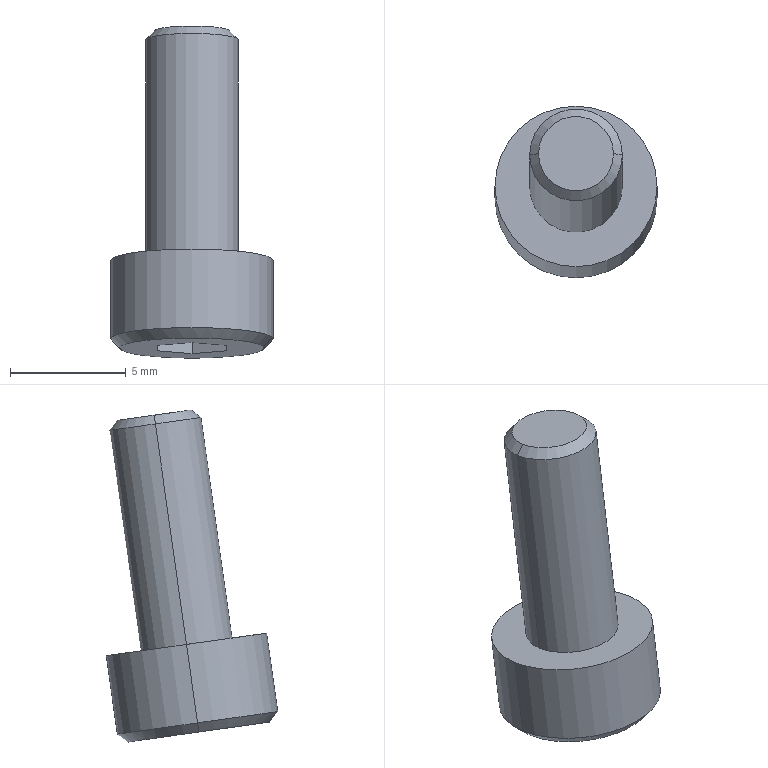Component | SolidWorks | 6G-TL06-Y-AxisMotorAssembly-2_6G-CPDW40-12-19-1_6G-CPDW40-12-19.stp-1_6G-M4-1 | 1 solid | 25 faces | box 7 x 7.41 x 14.34 mm | volume 253 mm3 | plane 15 | cone 6 | cylinder 4 | commonest cylinder face diameters 7 x2 4 x2
STEP:
#1=COLOUR_RGB('',0.7922,0.8196,0.9333);
#2=FILL_AREA_STYLE_COLOUR('',#1);
#3=FILL_AREA_STYLE('',(#2));
#4=SURFACE_STYLE_FILL_AREA(#3);
#5=SURFACE_SIDE_STYLE('',(#4));
#6=SURFACE_STYLE_USAGE(.BOTH.,#5);
#7=PRESENTATION_STYLE_ASSIGNMENT((#6));
#8=CARTESIAN_POINT('',(5.752,-0.6223,0.604));
#9=VERTEX_POINT('',#8);
#10=CARTESIAN_POINT('',(5.508,-0.6223,0.604));
#11=VERTEX_POINT('',#10);
#12=CARTESIAN_POINT('',(5.63,-0.6223,0.604));
#13=DIRECTION('',(0.,0.1396,0.9902));
#14=DIRECTION('',(1.,0.,0.));
#15=AXIS2_PLACEMENT_3D('',#12,#13,#14);
#16=CIRCLE('',#15,0.122);
#17=EDGE_CURVE('',#9,#11,#16,.T.);
#18=ORIENTED_EDGE('',*,*,#17,.T.);
#19=CARTESIAN_POINT('',(5.492,-0.6201,0.6196));
#20=VERTEX_POINT('',#19);
#21=CARTESIAN_POINT('',(5.508,-0.6223,0.604));
#22=DIRECTION('',(-0.7071,0.09872,0.7002));
#23=VECTOR('',#22,39.37);
#24=LINE('',#21,#23);
#25=EDGE_CURVE('',#11,#20,#24,.T.);
#26=ORIENTED_EDGE('',*,*,#25,.T.);
#27=CARTESIAN_POINT('',(5.768,-0.6201,0.6196));
#28=VERTEX_POINT('',#27);
#29=CARTESIAN_POINT('',(5.63,-0.6201,0.6196));
#30=DIRECTION('',(0.,0.1396,0.9902));
#31=DIRECTION('',(1.,0.,0.));
#32=AXIS2_PLACEMENT_3D('',#29,#30,#31);
#33=CIRCLE('',#32,0.1378);
#34=EDGE_CURVE('',#28,#20,#33,.T.);
#35=ORIENTED_EDGE('',*,*,#34,.F.);
#36=CARTESIAN_POINT('',(5.752,-0.6223,0.604));
#37=DIRECTION('',(0.7071,0.09872,0.7002));
#38=VECTOR('',#37,39.37);
#39=LINE('',#36,#38);
#40=EDGE_CURVE('',#9,#28,#39,.T.);
#41=ORIENTED_EDGE('',*,*,#40,.F.);
#42=EDGE_LOOP('',(#18,#26,#35,#41));
#43=FACE_OUTER_BOUND('',#42,.T.);
#44=CARTESIAN_POINT('',(5.63,-0.6223,0.604));
#45=DIRECTION('',(0.,0.1396,0.9902));
#46=DIRECTION('',(1.,0.,0.));
#47=AXIS2_PLACEMENT_3D('',#44,#45,#46);
#48=CONICAL_SURFACE('',#47,0.122,0.7854);
#49=ADVANCED_FACE('',(#43),#48,.T.);
#50=CARTESIAN_POINT('',(5.492,-0.6013,0.7529));
#51=VERTEX_POINT('',#50);
#52=CARTESIAN_POINT('',(5.768,-0.6013,0.7529));
#53=VERTEX_POINT('',#52);
#54=CARTESIAN_POINT('',(5.63,-0.6013,0.7529));
#55=DIRECTION('',(0.,0.1396,0.9902));
#56=DIRECTION('',(1.,0.,0.));
#57=AXIS2_PLACEMENT_3D('',#54,#55,#56);
#58=CIRCLE('',#57,0.1378);
#59=EDGE_CURVE('',#51,#53,#58,.T.);
#60=ORIENTED_EDGE('',*,*,#59,.F.);
#61=CARTESIAN_POINT('',(5.492,-0.5463,1.143));
#62=DIRECTION('',(0.,-0.1396,-0.9902));
#63=VECTOR('',#62,39.37);
#64=LINE('',#61,#63);
#65=EDGE_CURVE('',#51,#20,#64,.T.);
#66=ORIENTED_EDGE('',*,*,#65,.T.);
#67=CARTESIAN_POINT('',(5.63,-0.6201,0.6196));
#68=DIRECTION('',(0.,0.1396,0.9902));
#69=DIRECTION('',(1.,0.,0.));
#70=AXIS2_PLACEMENT_3D('',#67,#68,#69);
#71=CIRCLE('',#70,0.1378);
#72=EDGE_CURVE('',#20,#28,#71,.T.);
#73=ORIENTED_EDGE('',*,*,#72,.T.);
#74=CARTESIAN_POINT('',(5.768,-0.5463,1.143));
#75=DIRECTION('',(0.,-0.1396,-0.9902));
#76=VECTOR('',#75,39.37);
#77=LINE('',#74,#76);
#78=EDGE_CURVE('',#53,#28,#77,.T.);
#79=ORIENTED_EDGE('',*,*,#78,.F.);
#80=EDGE_LOOP('',(#60,#66,#73,#79));
#81=FACE_OUTER_BOUND('',#80,.T.);
#82=CARTESIAN_POINT('',(5.63,-0.5463,1.143));
#83=DIRECTION('',(0.,-0.1396,-0.9902));
#84=DIRECTION('',(1.,0.,0.));
#85=AXIS2_PLACEMENT_3D('',#82,#83,#84);
#86=CYLINDRICAL_SURFACE('',#85,0.1378);
#87=ADVANCED_FACE('',(#81),#86,.T.);
#88=CARTESIAN_POINT('',(5.551,-0.5484,1.128));
#89=VERTEX_POINT('',#88);
#90=CARTESIAN_POINT('',(5.709,-0.5484,1.128));
#91=VERTEX_POINT('',#90);
#92=CARTESIAN_POINT('',(5.63,-0.5484,1.128));
#93=DIRECTION('',(0.,0.1396,0.9902));
#94=DIRECTION('',(1.,0.,0.));
#95=AXIS2_PLACEMENT_3D('',#92,#93,#94);
#96=CIRCLE('',#95,0.07874);
#97=EDGE_CURVE('',#89,#91,#96,.T.);
#98=ORIENTED_EDGE('',*,*,#97,.F.);
#99=CARTESIAN_POINT('',(5.551,-0.6013,0.7529));
#100=VERTEX_POINT('',#99);
#101=CARTESIAN_POINT('',(5.551,-0.5463,1.143));
#102=DIRECTION('',(0.,-0.1396,-0.9902));
#103=VECTOR('',#102,39.37);
#104=LINE('',#101,#103);
#105=EDGE_CURVE('',#89,#100,#104,.T.);
#106=ORIENTED_EDGE('',*,*,#105,.T.);
#107=CARTESIAN_POINT('',(5.709,-0.6013,0.7529));
#108=VERTEX_POINT('',#107);
#109=CARTESIAN_POINT('',(5.63,-0.6013,0.7529));
#110=DIRECTION('',(0.,0.1396,0.9902));
#111=DIRECTION('',(1.,0.,0.));
#112=AXIS2_PLACEMENT_3D('',#109,#110,#111);
#113=CIRCLE('',#112,0.07874);
#114=EDGE_CURVE('',#100,#108,#113,.T.);
#115=ORIENTED_EDGE('',*,*,#114,.T.);
#116=CARTESIAN_POINT('',(5.709,-0.5463,1.143));
#117=DIRECTION('',(0.,-0.1396,-0.9902));
#118=VECTOR('',#117,39.37);
#119=LINE('',#116,#118);
#120=EDGE_CURVE('',#91,#108,#119,.T.);
#121=ORIENTED_EDGE('',*,*,#120,.F.);
#122=EDGE_LOOP('',(#98,#106,#115,#121));
#123=FACE_OUTER_BOUND('',#122,.T.);
#124=CARTESIAN_POINT('',(5.63,-0.5463,1.143));
#125=DIRECTION('',(0.,-0.1396,-0.9902));
#126=DIRECTION('',(1.,0.,0.));
#127=AXIS2_PLACEMENT_3D('',#124,#125,#126);
#128=CYLINDRICAL_SURFACE('',#127,0.07874);
#129=ADVANCED_FACE('',(#123),#128,.T.);
#130=CARTESIAN_POINT('',(5.694,-0.5463,1.143));
#131=VERTEX_POINT('',#130);
#132=CARTESIAN_POINT('',(5.566,-0.5463,1.143));
#133=VERTEX_POINT('',#132);
#134=CARTESIAN_POINT('',(5.63,-0.5463,1.143));
#135=DIRECTION('',(0.,0.1396,0.9902));
#136=DIRECTION('',(1.,0.,0.));
#137=AXIS2_PLACEMENT_3D('',#134,#135,#136);
#138=CIRCLE('',#137,0.06382);
#139=EDGE_CURVE('',#131,#133,#138,.T.);
#140=ORIENTED_EDGE('',*,*,#139,.F.);
#141=CARTESIAN_POINT('',(5.709,-0.5484,1.128));
#142=DIRECTION('',(0.7071,-0.09872,-0.7002));
#143=VECTOR('',#142,39.37);
#144=LINE('',#141,#143);
#145=EDGE_CURVE('',#131,#91,#144,.T.);
#146=ORIENTED_EDGE('',*,*,#145,.T.);
#147=CARTESIAN_POINT('',(5.63,-0.5484,1.128));
#148=DIRECTION('',(0.,0.1396,0.9902));
#149=DIRECTION('',(1.,0.,0.));
#150=AXIS2_PLACEMENT_3D('',#147,#148,#149);
#151=CIRCLE('',#150,0.07874);
#152=EDGE_CURVE('',#91,#89,#151,.T.);
#153=ORIENTED_EDGE('',*,*,#152,.T.);
#154=CARTESIAN_POINT('',(5.551,-0.5484,1.128));
#155=DIRECTION('',(-0.7071,-0.09872,-0.7002));
#156=VECTOR('',#155,39.37);
#157=LINE('',#154,#156);
#158=EDGE_CURVE('',#133,#89,#157,.T.);
#159=ORIENTED_EDGE('',*,*,#158,.F.);
#160=EDGE_LOOP('',(#140,#146,#153,#159));
#161=FACE_OUTER_BOUND('',#160,.T.);
#162=CARTESIAN_POINT('',(5.63,-0.5484,1.128));
#163=DIRECTION('',(0.,-0.1396,-0.9902));
#164=DIRECTION('',(-1.,0.,0.));
#165=AXIS2_PLACEMENT_3D('',#162,#163,#164);
#166=CONICAL_SURFACE('',#165,0.07874,0.7854);
#167=ADVANCED_FACE('',(#161),#166,.T.);
#168=CARTESIAN_POINT('',(5.63,-0.6065,0.7157));
#169=VERTEX_POINT('',#168);
#170=CARTESIAN_POINT('',(5.63,-0.6697,0.6902));
#171=VERTEX_POINT('',#170);
#172=CARTESIAN_POINT('',(5.63,-0.6697,0.6902));
#173=DIRECTION('',(0.,-0.9274,-0.3742));
#174=VECTOR('',#173,39.37);
#175=LINE('',#172,#174);
#176=EDGE_CURVE('',#169,#171,#175,.T.);
#177=ORIENTED_EDGE('',*,*,#176,.F.);
#178=CARTESIAN_POINT('',(5.63,-0.5528,0.6737));
#179=VERTEX_POINT('',#178);
#180=CARTESIAN_POINT('',(5.63,-0.5528,0.6737));
#181=DIRECTION('',(-0.,0.7877,-0.616));
#182=VECTOR('',#181,39.37);
#183=LINE('',#180,#182);
#184=EDGE_CURVE('',#169,#179,#183,.T.);
#185=ORIENTED_EDGE('',*,*,#184,.T.);
#186=CARTESIAN_POINT('',(5.659,-0.5606,0.6748));
#187=VERTEX_POINT('',#186);
#188=CARTESIAN_POINT('',(5.63,-0.6113,0.6819));
#189=DIRECTION('',(0.,-0.1396,-0.9902));
#190=DIRECTION('',(1.,0.,0.));
#191=AXIS2_PLACEMENT_3D('',#188,#189,#190);
#192=CIRCLE('',#191,0.05906);
#193=EDGE_CURVE('',#179,#187,#192,.T.);
#194=ORIENTED_EDGE('',*,*,#193,.T.);
#195=CARTESIAN_POINT('',(5.689,-0.6113,0.6819));
#196=VERTEX_POINT('',#195);
#197=CARTESIAN_POINT('',(5.63,-0.6113,0.6819));
#198=DIRECTION('',(0.,-0.1396,-0.9902));
#199=DIRECTION('',(1.,0.,0.));
#200=AXIS2_PLACEMENT_3D('',#197,#198,#199);
#201=CIRCLE('',#200,0.05906);
#202=EDGE_CURVE('',#187,#196,#201,.T.);
#203=ORIENTED_EDGE('',*,*,#202,.T.);
#204=CARTESIAN_POINT('',(5.659,-0.6619,0.6891));
#205=VERTEX_POINT('',#204);
#206=CARTESIAN_POINT('',(5.63,-0.6113,0.6819));
#207=DIRECTION('',(0.,-0.1396,-0.9902));
#208=DIRECTION('',(1.,0.,0.));
#209=AXIS2_PLACEMENT_3D('',#206,#207,#208);
#210=CIRCLE('',#209,0.05906);
#211=EDGE_CURVE('',#196,#205,#210,.T.);
#212=ORIENTED_EDGE('',*,*,#211,.T.);
#213=CARTESIAN_POINT('',(5.63,-0.6113,0.6819));
#214=DIRECTION('',(0.,-0.1396,-0.9902));
#215=DIRECTION('',(1.,0.,0.));
#216=AXIS2_PLACEMENT_3D('',#213,#214,#215);
#217=CIRCLE('',#216,0.05906);
#218=EDGE_CURVE('',#205,#171,#217,.T.);
#219=ORIENTED_EDGE('',*,*,#218,.T.);
#220=EDGE_LOOP('',(#177,#185,#194,#203,#212,#219));
#221=FACE_OUTER_BOUND('',#220,.T.);
#222=CARTESIAN_POINT('',(5.63,-0.6113,0.6819));
#223=DIRECTION('',(0.,-0.1396,-0.9902));
#224=DIRECTION('',(0.,-0.9902,0.1396));
#225=AXIS2_PLACEMENT_3D('',#222,#223,#224);
#226=CONICAL_SURFACE('',#225,0.05906,1.047);
#227=ADVANCED_FACE('',(#221),#226,.F.);
#228=ORIENTED_EDGE('',*,*,#184,.F.);
#229=ORIENTED_EDGE('',*,*,#176,.T.);
#230=CARTESIAN_POINT('',(5.6,-0.6619,0.6891));
#231=VERTEX_POINT('',#230);
#232=CARTESIAN_POINT('',(5.63,-0.6113,0.6819));
#233=DIRECTION('',(0.,-0.1396,-0.9902));
#234=DIRECTION('',(1.,0.,0.));
#235=AXIS2_PLACEMENT_3D('',#232,#233,#234);
#236=CIRCLE('',#235,0.05906);
#237=EDGE_CURVE('',#171,#231,#236,.T.);
#238=ORIENTED_EDGE('',*,*,#237,.T.);
#239=CARTESIAN_POINT('',(5.571,-0.6113,0.6819));
#240=VERTEX_POINT('',#239);
#241=CARTESIAN_POINT('',(5.63,-0.6113,0.6819));
#242=DIRECTION('',(0.,-0.1396,-0.9902));
#243=DIRECTION('',(1.,0.,0.));
#244=AXIS2_PLACEMENT_3D('',#241,#242,#243);
#245=CIRCLE('',#244,0.05906);
#246=EDGE_CURVE('',#231,#240,#245,.T.);
#247=ORIENTED_EDGE('',*,*,#246,.T.);
#248=CARTESIAN_POINT('',(5.6,-0.5606,0.6748));
#249=VERTEX_POINT('',#248);
#250=CARTESIAN_POINT('',(5.63,-0.6113,0.6819));
#251=DIRECTION('',(0.,-0.1396,-0.9902));
#252=DIRECTION('',(1.,0.,0.));
#253=AXIS2_PLACEMENT_3D('',#250,#251,#252);
#254=CIRCLE('',#253,0.05906);
#255=EDGE_CURVE('',#240,#249,#254,.T.);
#256=ORIENTED_EDGE('',*,*,#255,.T.);
#257=CARTESIAN_POINT('',(5.63,-0.6113,0.6819));
#258=DIRECTION('',(0.,-0.1396,-0.9902));
#259=DIRECTION('',(1.,0.,0.));
#260=AXIS2_PLACEMENT_3D('',#257,#258,#259);
#261=CIRCLE('',#260,0.05906);
#262=EDGE_CURVE('',#249,#179,#261,.T.);
#263=ORIENTED_EDGE('',*,*,#262,.T.);
#264=EDGE_LOOP('',(#228,#229,#238,#247,#256,#263));
#265=FACE_OUTER_BOUND('',#264,.T.);
#266=CARTESIAN_POINT('',(5.63,-0.6113,0.6819));
#267=DIRECTION('',(0.,-0.1396,-0.9902));
#268=DIRECTION('',(0.,-0.9902,0.1396));
#269=AXIS2_PLACEMENT_3D('',#266,#267,#268);
#270=CONICAL_SURFACE('',#269,0.05906,1.047);
#271=ADVANCED_FACE('',(#265),#270,.F.);
#272=ORIENTED_EDGE('',*,*,#262,.F.);
#273=CARTESIAN_POINT('',(5.63,-0.5437,0.6724));
#274=VERTEX_POINT('',#273);
#275=CARTESIAN_POINT('',(5.63,-0.5437,0.6724));
#276=DIRECTION('',(-0.866,-0.4951,0.06981));
#277=VECTOR('',#276,39.37);
#278=LINE('',#275,#277);
#279=EDGE_CURVE('',#274,#249,#278,.T.);
#280=ORIENTED_EDGE('',*,*,#279,.F.);
#281=CARTESIAN_POINT('',(5.689,-0.5775,0.6772));
#282=DIRECTION('',(-0.866,0.4951,-0.06981));
#283=VECTOR('',#282,39.37);
#284=LINE('',#281,#283);
#285=EDGE_CURVE('',#187,#274,#284,.T.);
#286=ORIENTED_EDGE('',*,*,#285,.F.);
#287=ORIENTED_EDGE('',*,*,#193,.F.);
#288=EDGE_LOOP('',(#272,#280,#286,#287));
#289=FACE_OUTER_BOUND('',#288,.T.);
#290=CARTESIAN_POINT('',(5.63,-0.6113,0.6819));
#291=DIRECTION('',(0.,0.1396,0.9902));
#292=DIRECTION('',(0.,0.9902,-0.1396));
#293=AXIS2_PLACEMENT_3D('',#290,#291,#292);
#294=PLANE('',#293);
#295=ADVANCED_FACE('',(#289),#294,.F.);
#296=ORIENTED_EDGE('',*,*,#211,.F.);
#297=CARTESIAN_POINT('',(5.689,-0.645,0.6867));
#298=VERTEX_POINT('',#297);
#299=CARTESIAN_POINT('',(5.689,-0.645,0.6867));
#300=DIRECTION('',(0.,0.9902,-0.1396));
#301=VECTOR('',#300,39.37);
#302=LINE('',#299,#301);
#303=EDGE_CURVE('',#298,#196,#302,.T.);
#304=ORIENTED_EDGE('',*,*,#303,.F.);
#305=CARTESIAN_POINT('',(5.63,-0.6788,0.6915));
#306=DIRECTION('',(0.866,0.4951,-0.06981));
#307=VECTOR('',#306,39.37);
#308=LINE('',#305,#307);
#309=EDGE_CURVE('',#205,#298,#308,.T.);
#310=ORIENTED_EDGE('',*,*,#309,.F.);
#311=EDGE_LOOP('',(#296,#304,#310));
#312=FACE_OUTER_BOUND('',#311,.T.);
#313=CARTESIAN_POINT('',(5.63,-0.6113,0.6819));
#314=DIRECTION('',(0.,0.1396,0.9902));
#315=DIRECTION('',(0.,0.9902,-0.1396));
#316=AXIS2_PLACEMENT_3D('',#313,#314,#315);
#317=PLANE('',#316);
#318=ADVANCED_FACE('',(#312),#317,.F.);
#319=ORIENTED_EDGE('',*,*,#255,.F.);
#320=CARTESIAN_POINT('',(5.571,-0.5775,0.6772));
#321=VERTEX_POINT('',#320);
#322=CARTESIAN_POINT('',(5.571,-0.5775,0.6772));
#323=DIRECTION('',(0.,-0.9902,0.1396));
#324=VECTOR('',#323,39.37);
#325=LINE('',#322,#324);
#326=EDGE_CURVE('',#321,#240,#325,.T.);
#327=ORIENTED_EDGE('',*,*,#326,.F.);
#328=CARTESIAN_POINT('',(5.63,-0.5437,0.6724));
#329=DIRECTION('',(-0.866,-0.4951,0.06981));
#330=VECTOR('',#329,39.37);
#331=LINE('',#328,#330);
#332=EDGE_CURVE('',#249,#321,#331,.T.);
#333=ORIENTED_EDGE('',*,*,#332,.F.);
#334=EDGE_LOOP('',(#319,#327,#333));
#335=FACE_OUTER_BOUND('',#334,.T.);
#336=CARTESIAN_POINT('',(5.63,-0.6113,0.6819));
#337=DIRECTION('',(0.,0.1396,0.9902));
#338=DIRECTION('',(0.,0.9902,-0.1396));
#339=AXIS2_PLACEMENT_3D('',#336,#337,#338);
#340=PLANE('',#339);
#341=ADVANCED_FACE('',(#335),#340,.F.);
#342=ORIENTED_EDGE('',*,*,#218,.F.);
#343=CARTESIAN_POINT('',(5.63,-0.6788,0.6915));
#344=VERTEX_POINT('',#343);
#345=CARTESIAN_POINT('',(5.63,-0.6788,0.6915));
#346=DIRECTION('',(0.866,0.4951,-0.06981));
#347=VECTOR('',#346,39.37);
#348=LINE('',#345,#347);
#349=EDGE_CURVE('',#344,#205,#348,.T.);
#350=ORIENTED_EDGE('',*,*,#349,.F.);
#351=CARTESIAN_POINT('',(5.571,-0.645,0.6867));
#352=DIRECTION('',(0.866,-0.4951,0.06981));
#353=VECTOR('',#352,39.37);
#354=LINE('',#351,#353);
#355=EDGE_CURVE('',#231,#344,#354,.T.);
#356=ORIENTED_EDGE('',*,*,#355,.F.);
#357=ORIENTED_EDGE('',*,*,#237,.F.);
#358=EDGE_LOOP('',(#342,#350,#356,#357));
#359=FACE_OUTER_BOUND('',#358,.T.);
#360=CARTESIAN_POINT('',(5.63,-0.6113,0.6819));
#361=DIRECTION('',(0.,0.1396,0.9902));
#362=DIRECTION('',(0.,0.9902,-0.1396));
#363=AXIS2_PLACEMENT_3D('',#360,#361,#362);
#364=PLANE('',#363);
#365=ADVANCED_FACE('',(#359),#364,.F.);
#366=ORIENTED_EDGE('',*,*,#246,.F.);
#367=CARTESIAN_POINT('',(5.571,-0.645,0.6867));
#368=VERTEX_POINT('',#367);
#369=CARTESIAN_POINT('',(5.571,-0.645,0.6867));
#370=DIRECTION('',(0.866,-0.4951,0.06981));
#371=VECTOR('',#370,39.37);
#372=LINE('',#369,#371);
#373=EDGE_CURVE('',#368,#231,#372,.T.);
#374=ORIENTED_EDGE('',*,*,#373,.F.);
#375=CARTESIAN_POINT('',(5.571,-0.5775,0.6772));
#376=DIRECTION('',(0.,-0.9902,0.1396));
#377=VECTOR('',#376,39.37);
#378=LINE('',#375,#377);
#379=EDGE_CURVE('',#240,#368,#378,.T.);
#380=ORIENTED_EDGE('',*,*,#379,.F.);
#381=EDGE_LOOP('',(#366,#374,#380));
#382=FACE_OUTER_BOUND('',#381,.T.);
#383=CARTESIAN_POINT('',(5.63,-0.6113,0.6819));
#384=DIRECTION('',(0.,0.1396,0.9902));
#385=DIRECTION('',(0.,0.9902,-0.1396));
#386=AXIS2_PLACEMENT_3D('',#383,#384,#385);
#387=PLANE('',#386);
#388=ADVANCED_FACE('',(#382),#387,.F.);
#389=ORIENTED_EDGE('',*,*,#202,.F.);
#390=CARTESIAN_POINT('',(5.689,-0.5775,0.6772));
#391=VERTEX_POINT('',#390);
#392=CARTESIAN_POINT('',(5.689,-0.5775,0.6772));
#393=DIRECTION('',(-0.866,0.4951,-0.06981));
#394=VECTOR('',#393,39.37);
#395=LINE('',#392,#394);
#396=EDGE_CURVE('',#391,#187,#395,.T.);
#397=ORIENTED_EDGE('',*,*,#396,.F.);
#398=CARTESIAN_POINT('',(5.689,-0.645,0.6867));
#399=DIRECTION('',(0.,0.9902,-0.1396));
#400=VECTOR('',#399,39.37);
#401=LINE('',#398,#400);
#402=EDGE_CURVE('',#196,#391,#401,.T.);
#403=ORIENTED_EDGE('',*,*,#402,.F.);
#404=EDGE_LOOP('',(#389,#397,#403));
#405=FACE_OUTER_BOUND('',#404,.T.);
#406=CARTESIAN_POINT('',(5.63,-0.6113,0.6819));
#407=DIRECTION('',(0.,0.1396,0.9902));
#408=DIRECTION('',(0.,0.9902,-0.1396));
#409=AXIS2_PLACEMENT_3D('',#406,#407,#408);
#410=PLANE('',#409);
#411=ADVANCED_FACE('',(#405),#410,.F.);
#412=CARTESIAN_POINT('',(5.63,-0.5547,0.5945));
#413=VERTEX_POINT('',#412);
#414=CARTESIAN_POINT('',(5.571,-0.5885,0.5992));
#415=VERTEX_POINT('',#414);
#416=CARTESIAN_POINT('',(5.63,-0.5547,0.5945));
#417=DIRECTION('',(-0.866,-0.4951,0.06981));
#418=VECTOR('',#417,39.37);
#419=LINE('',#416,#418);
#420=EDGE_CURVE('',#413,#415,#419,.T.);
#421=ORIENTED_EDGE('',*,*,#420,.F.);
#422=CARTESIAN_POINT('',(5.63,-0.5437,0.6724));
#423=DIRECTION('',(0.,-0.1396,-0.9902));
#424=VECTOR('',#423,39.37);
#425=LINE('',#422,#424);
#426=EDGE_CURVE('',#274,#413,#425,.T.);
#427=ORIENTED_EDGE('',*,*,#426,.F.);
#428=ORIENTED_EDGE('',*,*,#279,.T.);
#429=ORIENTED_EDGE('',*,*,#332,.T.);
#430=CARTESIAN_POINT('',(5.571,-0.5775,0.6772));
#431=DIRECTION('',(0.,-0.1396,-0.9902));
#432=VECTOR('',#431,39.37);
#433=LINE('',#430,#432);
#434=EDGE_CURVE('',#321,#415,#433,.T.);
#435=ORIENTED_EDGE('',*,*,#434,.T.);
#436=EDGE_LOOP('',(#421,#427,#428,#429,#435));
#437=FACE_OUTER_BOUND('',#436,.T.);
#438=CARTESIAN_POINT('',(5.63,-0.5437,0.6724));
#439=DIRECTION('',(0.5,-0.8575,0.1209));
#440=DIRECTION('',(0.866,0.4951,-0.06981));
#441=AXIS2_PLACEMENT_3D('',#438,#439,#440);
#442=PLANE('',#441);
#443=ADVANCED_FACE('',(#437),#442,.T.);
#444=CARTESIAN_POINT('',(5.689,-0.5885,0.5992));
#445=VERTEX_POINT('',#444);
#446=CARTESIAN_POINT('',(5.689,-0.5885,0.5992));
#447=DIRECTION('',(-0.866,0.4951,-0.06981));
#448=VECTOR('',#447,39.37);
#449=LINE('',#446,#448);
#450=EDGE_CURVE('',#445,#413,#449,.T.);
#451=ORIENTED_EDGE('',*,*,#450,.F.);
#452=CARTESIAN_POINT('',(5.689,-0.5775,0.6772));
#453=DIRECTION('',(0.,-0.1396,-0.9902));
#454=VECTOR('',#453,39.37);
#455=LINE('',#452,#454);
#456=EDGE_CURVE('',#391,#445,#455,.T.);
#457=ORIENTED_EDGE('',*,*,#456,.F.);
#458=ORIENTED_EDGE('',*,*,#396,.T.);
#459=ORIENTED_EDGE('',*,*,#285,.T.);
#460=ORIENTED_EDGE('',*,*,#426,.T.);
#461=EDGE_LOOP('',(#451,#457,#458,#459,#460));
#462=FACE_OUTER_BOUND('',#461,.T.);
#463=CARTESIAN_POINT('',(5.689,-0.5775,0.6772));
#464=DIRECTION('',(-0.5,-0.8575,0.1209));
#465=DIRECTION('',(0.,-0.1396,-0.9902));
#466=AXIS2_PLACEMENT_3D('',#463,#464,#465);
#467=PLANE('',#466);
#468=ADVANCED_FACE('',(#462),#467,.T.);
#469=CARTESIAN_POINT('',(5.689,-0.656,0.6087));
#470=VERTEX_POINT('',#469);
#471=CARTESIAN_POINT('',(5.689,-0.656,0.6087));
#472=DIRECTION('',(0.,0.9902,-0.1396));
#473=VECTOR('',#472,39.37);
#474=LINE('',#471,#473);
#475=EDGE_CURVE('',#470,#445,#474,.T.);
#476=ORIENTED_EDGE('',*,*,#475,.F.);
#477=CARTESIAN_POINT('',(5.689,-0.645,0.6867));
#478=DIRECTION('',(0.,-0.1396,-0.9902));
#479=VECTOR('',#478,39.37);
#480=LINE('',#477,#479);
#481=EDGE_CURVE('',#298,#470,#480,.T.);
#482=ORIENTED_EDGE('',*,*,#481,.F.);
#483=ORIENTED_EDGE('',*,*,#303,.T.);
#484=ORIENTED_EDGE('',*,*,#402,.T.);
#485=ORIENTED_EDGE('',*,*,#456,.T.);
#486=EDGE_LOOP('',(#476,#482,#483,#484,#485));
#487=FACE_OUTER_BOUND('',#486,.T.);
#488=CARTESIAN_POINT('',(5.689,-0.645,0.6867));
#489=DIRECTION('',(-1.,0.,0.));
#490=DIRECTION('',(0.,0.1396,0.9902));
#491=AXIS2_PLACEMENT_3D('',#488,#489,#490);
#492=PLANE('',#491);
#493=ADVANCED_FACE('',(#487),#492,.T.);
#494=CARTESIAN_POINT('',(5.63,-0.6898,0.6135));
#495=VERTEX_POINT('',#494);
#496=CARTESIAN_POINT('',(5.63,-0.6898,0.6135));
#497=DIRECTION('',(0.866,0.4951,-0.06981));
#498=VECTOR('',#497,39.37);
#499=LINE('',#496,#498);
#500=EDGE_CURVE('',#495,#470,#499,.T.);
#501=ORIENTED_EDGE('',*,*,#500,.F.);
#502=CARTESIAN_POINT('',(5.63,-0.6788,0.6915));
#503=DIRECTION('',(0.,-0.1396,-0.9902));
#504=VECTOR('',#503,39.37);
#505=LINE('',#502,#504);
#506=EDGE_CURVE('',#344,#495,#505,.T.);
#507=ORIENTED_EDGE('',*,*,#506,.F.);
#508=ORIENTED_EDGE('',*,*,#349,.T.);
#509=ORIENTED_EDGE('',*,*,#309,.T.);
#510=ORIENTED_EDGE('',*,*,#481,.T.);
#511=EDGE_LOOP('',(#501,#507,#508,#509,#510));
#512=FACE_OUTER_BOUND('',#511,.T.);
#513=CARTESIAN_POINT('',(5.63,-0.6788,0.6915));
#514=DIRECTION('',(-0.5,0.8575,-0.1209));
#515=DIRECTION('',(0.,0.1396,0.9902));
#516=AXIS2_PLACEMENT_3D('',#513,#514,#515);
#517=PLANE('',#516);
#518=ADVANCED_FACE('',(#512),#517,.T.);
#519=CARTESIAN_POINT('',(5.571,-0.656,0.6087));
#520=VERTEX_POINT('',#519);
#521=CARTESIAN_POINT('',(5.571,-0.656,0.6087));
#522=DIRECTION('',(0.866,-0.4951,0.06981));
#523=VECTOR('',#522,39.37);
#524=LINE('',#521,#523);
#525=EDGE_CURVE('',#520,#495,#524,.T.);
#526=ORIENTED_EDGE('',*,*,#525,.F.);
#527=CARTESIAN_POINT('',(5.571,-0.645,0.6867));
#528=DIRECTION('',(0.,-0.1396,-0.9902));
#529=VECTOR('',#528,39.37);
#530=LINE('',#527,#529);
#531=EDGE_CURVE('',#368,#520,#530,.T.);
#532=ORIENTED_EDGE('',*,*,#531,.F.);
#533=ORIENTED_EDGE('',*,*,#373,.T.);
#534=ORIENTED_EDGE('',*,*,#355,.T.);
#535=ORIENTED_EDGE('',*,*,#506,.T.);
#536=EDGE_LOOP('',(#526,#532,#533,#534,#535));
#537=FACE_OUTER_BOUND('',#536,.T.);
#538=CARTESIAN_POINT('',(5.571,-0.645,0.6867));
#539=DIRECTION('',(0.5,0.8575,-0.1209));
#540=DIRECTION('',(0.,-0.1396,-0.9902));
#541=AXIS2_PLACEMENT_3D('',#538,#539,#540);
#542=PLANE('',#541);
#543=ADVANCED_FACE('',(#537),#542,.T.);
#544=CARTESIAN_POINT('',(5.571,-0.5885,0.5992));
#545=DIRECTION('',(0.,-0.9902,0.1396));
#546=VECTOR('',#545,39.37);
#547=LINE('',#544,#546);
#548=EDGE_CURVE('',#415,#520,#547,.T.);
#549=ORIENTED_EDGE('',*,*,#548,.F.);
#550=ORIENTED_EDGE('',*,*,#434,.F.);
#551=ORIENTED_EDGE('',*,*,#326,.T.);
#552=ORIENTED_EDGE('',*,*,#379,.T.);
#553=ORIENTED_EDGE('',*,*,#531,.T.);
#554=EDGE_LOOP('',(#549,#550,#551,#552,#553));
#555=FACE_OUTER_BOUND('',#554,.T.);
#556=CARTESIAN_POINT('',(5.571,-0.5775,0.6772));
#557=DIRECTION('',(1.,0.,0.));
#558=DIRECTION('',(0.,-0.9902,0.1396));
#559=AXIS2_PLACEMENT_3D('',#556,#557,#558);
#560=PLANE('',#559);
#561=ADVANCED_FACE('',(#555),#560,.T.);
#562=CARTESIAN_POINT('',(5.63,-0.5463,1.143));
#563=DIRECTION('',(0.,0.1396,0.9902));
#564=DIRECTION('',(1.,0.,0.));
#565=AXIS2_PLACEMENT_3D('',#562,#563,#564);
#566=CIRCLE('',#565,0.06382);
#567=EDGE_CURVE('',#133,#131,#566,.T.);
#568=ORIENTED_EDGE('',*,*,#567,.T.);
#569=ORIENTED_EDGE('',*,*,#139,.T.);
#570=EDGE_LOOP('',(#568,#569));
#571=FACE_OUTER_BOUND('',#570,.T.);
#572=CARTESIAN_POINT('',(5.63,-0.4831,1.134));
#573=DIRECTION('',(0.,-0.1396,-0.9902));
#574=DIRECTION('',(-1.,0.,0.));
#575=AXIS2_PLACEMENT_3D('',#572,#573,#574);
#576=PLANE('',#575);
#577=ADVANCED_FACE('',(#571),#576,.F.);
#578=ORIENTED_EDGE('',*,*,#145,.F.);
#579=ORIENTED_EDGE('',*,*,#567,.F.);
#580=ORIENTED_EDGE('',*,*,#158,.T.);
#581=ORIENTED_EDGE('',*,*,#97,.T.);
#582=EDGE_LOOP('',(#578,#579,#580,#581));
#583=FACE_OUTER_BOUND('',#582,.T.);
#584=CARTESIAN_POINT('',(5.63,-0.5484,1.128));
#585=DIRECTION('',(0.,-0.1396,-0.9902));
#586=DIRECTION('',(-1.,0.,0.));
#587=AXIS2_PLACEMENT_3D('',#584,#585,#586);
#588=CONICAL_SURFACE('',#587,0.07874,0.7854);
#589=ADVANCED_FACE('',(#583),#588,.T.);
#590=ORIENTED_EDGE('',*,*,#105,.F.);
#591=ORIENTED_EDGE('',*,*,#152,.F.);
#592=ORIENTED_EDGE('',*,*,#120,.T.);
#593=CARTESIAN_POINT('',(5.63,-0.6013,0.7529));
#594=DIRECTION('',(0.,0.1396,0.9902));
#595=DIRECTION('',(1.,0.,0.));
#596=AXIS2_PLACEMENT_3D('',#593,#594,#595);
#597=CIRCLE('',#596,0.07874);
#598=EDGE_CURVE('',#108,#100,#597,.T.);
#599=ORIENTED_EDGE('',*,*,#598,.T.);
#600=EDGE_LOOP('',(#590,#591,#592,#599));
#601=FACE_OUTER_BOUND('',#600,.T.);
#602=CARTESIAN_POINT('',(5.63,-0.5463,1.143));
#603=DIRECTION('',(0.,-0.1396,-0.9902));
#604=DIRECTION('',(1.,0.,0.));
#605=AXIS2_PLACEMENT_3D('',#602,#603,#604);
#606=CYLINDRICAL_SURFACE('',#605,0.07874);
#607=ADVANCED_FACE('',(#601),#606,.T.);
#608=CARTESIAN_POINT('',(5.63,-0.6013,0.7529));
#609=DIRECTION('',(0.,0.1396,0.9902));
#610=DIRECTION('',(1.,0.,0.));
#611=AXIS2_PLACEMENT_3D('',#608,#609,#610);
#612=CIRCLE('',#611,0.1378);
#613=EDGE_CURVE('',#53,#51,#612,.T.);
#614=ORIENTED_EDGE('',*,*,#613,.T.);
#615=ORIENTED_EDGE('',*,*,#59,.T.);
#616=EDGE_LOOP('',(#614,#615));
#617=FACE_OUTER_BOUND('',#616,.T.);
#618=ORIENTED_EDGE('',*,*,#598,.F.);
#619=ORIENTED_EDGE('',*,*,#114,.F.);
#620=EDGE_LOOP('',(#618,#619));
#621=FACE_BOUND('',#620,.T.);
#622=CARTESIAN_POINT('',(5.63,-0.4648,0.7337));
#623=DIRECTION('',(0.,-0.1396,-0.9902));
#624=DIRECTION('',(-1.,0.,0.));
#625=AXIS2_PLACEMENT_3D('',#622,#623,#624);
#626=PLANE('',#625);
#627=ADVANCED_FACE('',(#617,#621),#626,.F.);
#628=ORIENTED_EDGE('',*,*,#65,.F.);
#629=ORIENTED_EDGE('',*,*,#613,.F.);
#630=ORIENTED_EDGE('',*,*,#78,.T.);
#631=ORIENTED_EDGE('',*,*,#34,.T.);
#632=EDGE_LOOP('',(#628,#629,#630,#631));
#633=FACE_OUTER_BOUND('',#632,.T.);
#634=CARTESIAN_POINT('',(5.63,-0.5463,1.143));
#635=DIRECTION('',(0.,-0.1396,-0.9902));
#636=DIRECTION('',(1.,0.,0.));
#637=AXIS2_PLACEMENT_3D('',#634,#635,#636);
#638=CYLINDRICAL_SURFACE('',#637,0.1378);
#639=ADVANCED_FACE('',(#633),#638,.T.);
#640=ORIENTED_EDGE('',*,*,#25,.F.);
#641=CARTESIAN_POINT('',(5.63,-0.6223,0.604));
#642=DIRECTION('',(0.,0.1396,0.9902));
#643=DIRECTION('',(1.,0.,0.));
#644=AXIS2_PLACEMENT_3D('',#641,#642,#643);
#645=CIRCLE('',#644,0.122);
#646=EDGE_CURVE('',#11,#9,#645,.T.);
#647=ORIENTED_EDGE('',*,*,#646,.T.);
#648=ORIENTED_EDGE('',*,*,#40,.T.);
#649=ORIENTED_EDGE('',*,*,#72,.F.);
#650=EDGE_LOOP('',(#640,#647,#648,#649));
#651=FACE_OUTER_BOUND('',#650,.T.);
#652=CARTESIAN_POINT('',(5.63,-0.6223,0.604));
#653=DIRECTION('',(0.,0.1396,0.9902));
#654=DIRECTION('',(1.,0.,0.));
#655=AXIS2_PLACEMENT_3D('',#652,#653,#654);
#656=CONICAL_SURFACE('',#655,0.122,0.7854);
#657=ADVANCED_FACE('',(#651),#656,.T.);
#658=ORIENTED_EDGE('',*,*,#17,.F.);
#659=ORIENTED_EDGE('',*,*,#646,.F.);
#660=EDGE_LOOP('',(#658,#659));
#661=FACE_OUTER_BOUND('',#660,.T.);
#662=ORIENTED_EDGE('',*,*,#548,.T.);
#663=ORIENTED_EDGE('',*,*,#525,.T.);
#664=ORIENTED_EDGE('',*,*,#500,.T.);
#665=ORIENTED_EDGE('',*,*,#475,.T.);
#666=ORIENTED_EDGE('',*,*,#450,.T.);
#667=ORIENTED_EDGE('',*,*,#420,.T.);
#668=EDGE_LOOP('',(#662,#663,#664,#665,#666,#667));
#669=FACE_BOUND('',#668,.T.);
#670=CARTESIAN_POINT('',(5.63,-0.6223,0.604));
#671=DIRECTION('',(0.,0.1396,0.9902));
#672=DIRECTION('',(0.,0.9902,-0.1396));
#673=AXIS2_PLACEMENT_3D('',#670,#671,#672);
#674=PLANE('',#673);
#675=ADVANCED_FACE('',(#661,#669),#674,.F.);
#676=CLOSED_SHELL('',(#49,#87,#129,#167,#227,#271,#295,#318,#341,#365,#388,#411,#443,#468,#493,#518,#543,#561,#577,#589,#607,#627,#639,#657,#675));
#677=MANIFOLD_SOLID_BREP('',#676);
#678=STYLED_ITEM('',(#7),#677);
#679=PRESENTATION_LAYER_ASSIGNMENT('','',(#678));
#680=(LENGTH_UNIT()NAMED_UNIT(*)SI_UNIT($,.METRE.));
#681=LENGTH_MEASURE_WITH_UNIT(LENGTH_MEASURE(0.0254),#680);
#682=DIMENSIONAL_EXPONENTS(1.,0.,0.,0.,0.,0.,0.);
#683=(CONVERSION_BASED_UNIT('',#681)LENGTH_UNIT()NAMED_UNIT(#682));
#684=UNCERTAINTY_MEASURE_WITH_UNIT(LENGTH_MEASURE(0.00001),#683,'','');
#685=(NAMED_UNIT(*)PLANE_ANGLE_UNIT()SI_UNIT($,.RADIAN.));
#686=(NAMED_UNIT(*)SI_UNIT($,.STERADIAN.)SOLID_ANGLE_UNIT());
#687=(GEOMETRIC_REPRESENTATION_CONTEXT(3)GLOBAL_UNCERTAINTY_ASSIGNED_CONTEXT((#684))GLOBAL_UNIT_ASSIGNED_CONTEXT((#683,#685,#686))REPRESENTATION_CONTEXT('',''));
#688=MECHANICAL_DESIGN_GEOMETRIC_PRESENTATION_REPRESENTATION('',(#678),#687);
#689=CARTESIAN_POINT('',(0.,0.,0.));
#690=DIRECTION('',(0.,0.,1.));
#691=DIRECTION('',(1.,0.,0.));
#692=AXIS2_PLACEMENT_3D('',#689,#690,#691);
#693=(LENGTH_UNIT()NAMED_UNIT(*)SI_UNIT($,.METRE.));
#694=LENGTH_MEASURE_WITH_UNIT(LENGTH_MEASURE(0.0254),#693);
#695=DIMENSIONAL_EXPONENTS(1.,0.,0.,0.,0.,0.,0.);
#696=(CONVERSION_BASED_UNIT('',#694)LENGTH_UNIT()NAMED_UNIT(#695));
#697=UNCERTAINTY_MEASURE_WITH_UNIT(LENGTH_MEASURE(0.00001),#696,'','');
#698=(NAMED_UNIT(*)PLANE_ANGLE_UNIT()SI_UNIT($,.RADIAN.));
#699=(NAMED_UNIT(*)SI_UNIT($,.STERADIAN.)SOLID_ANGLE_UNIT());
#700=(GEOMETRIC_REPRESENTATION_CONTEXT(3)GLOBAL_UNCERTAINTY_ASSIGNED_CONTEXT((#697))GLOBAL_UNIT_ASSIGNED_CONTEXT((#696,#698,#699))REPRESENTATION_CONTEXT('',''));
#701=ADVANCED_BREP_SHAPE_REPRESENTATION('',(#677,#692),#700);